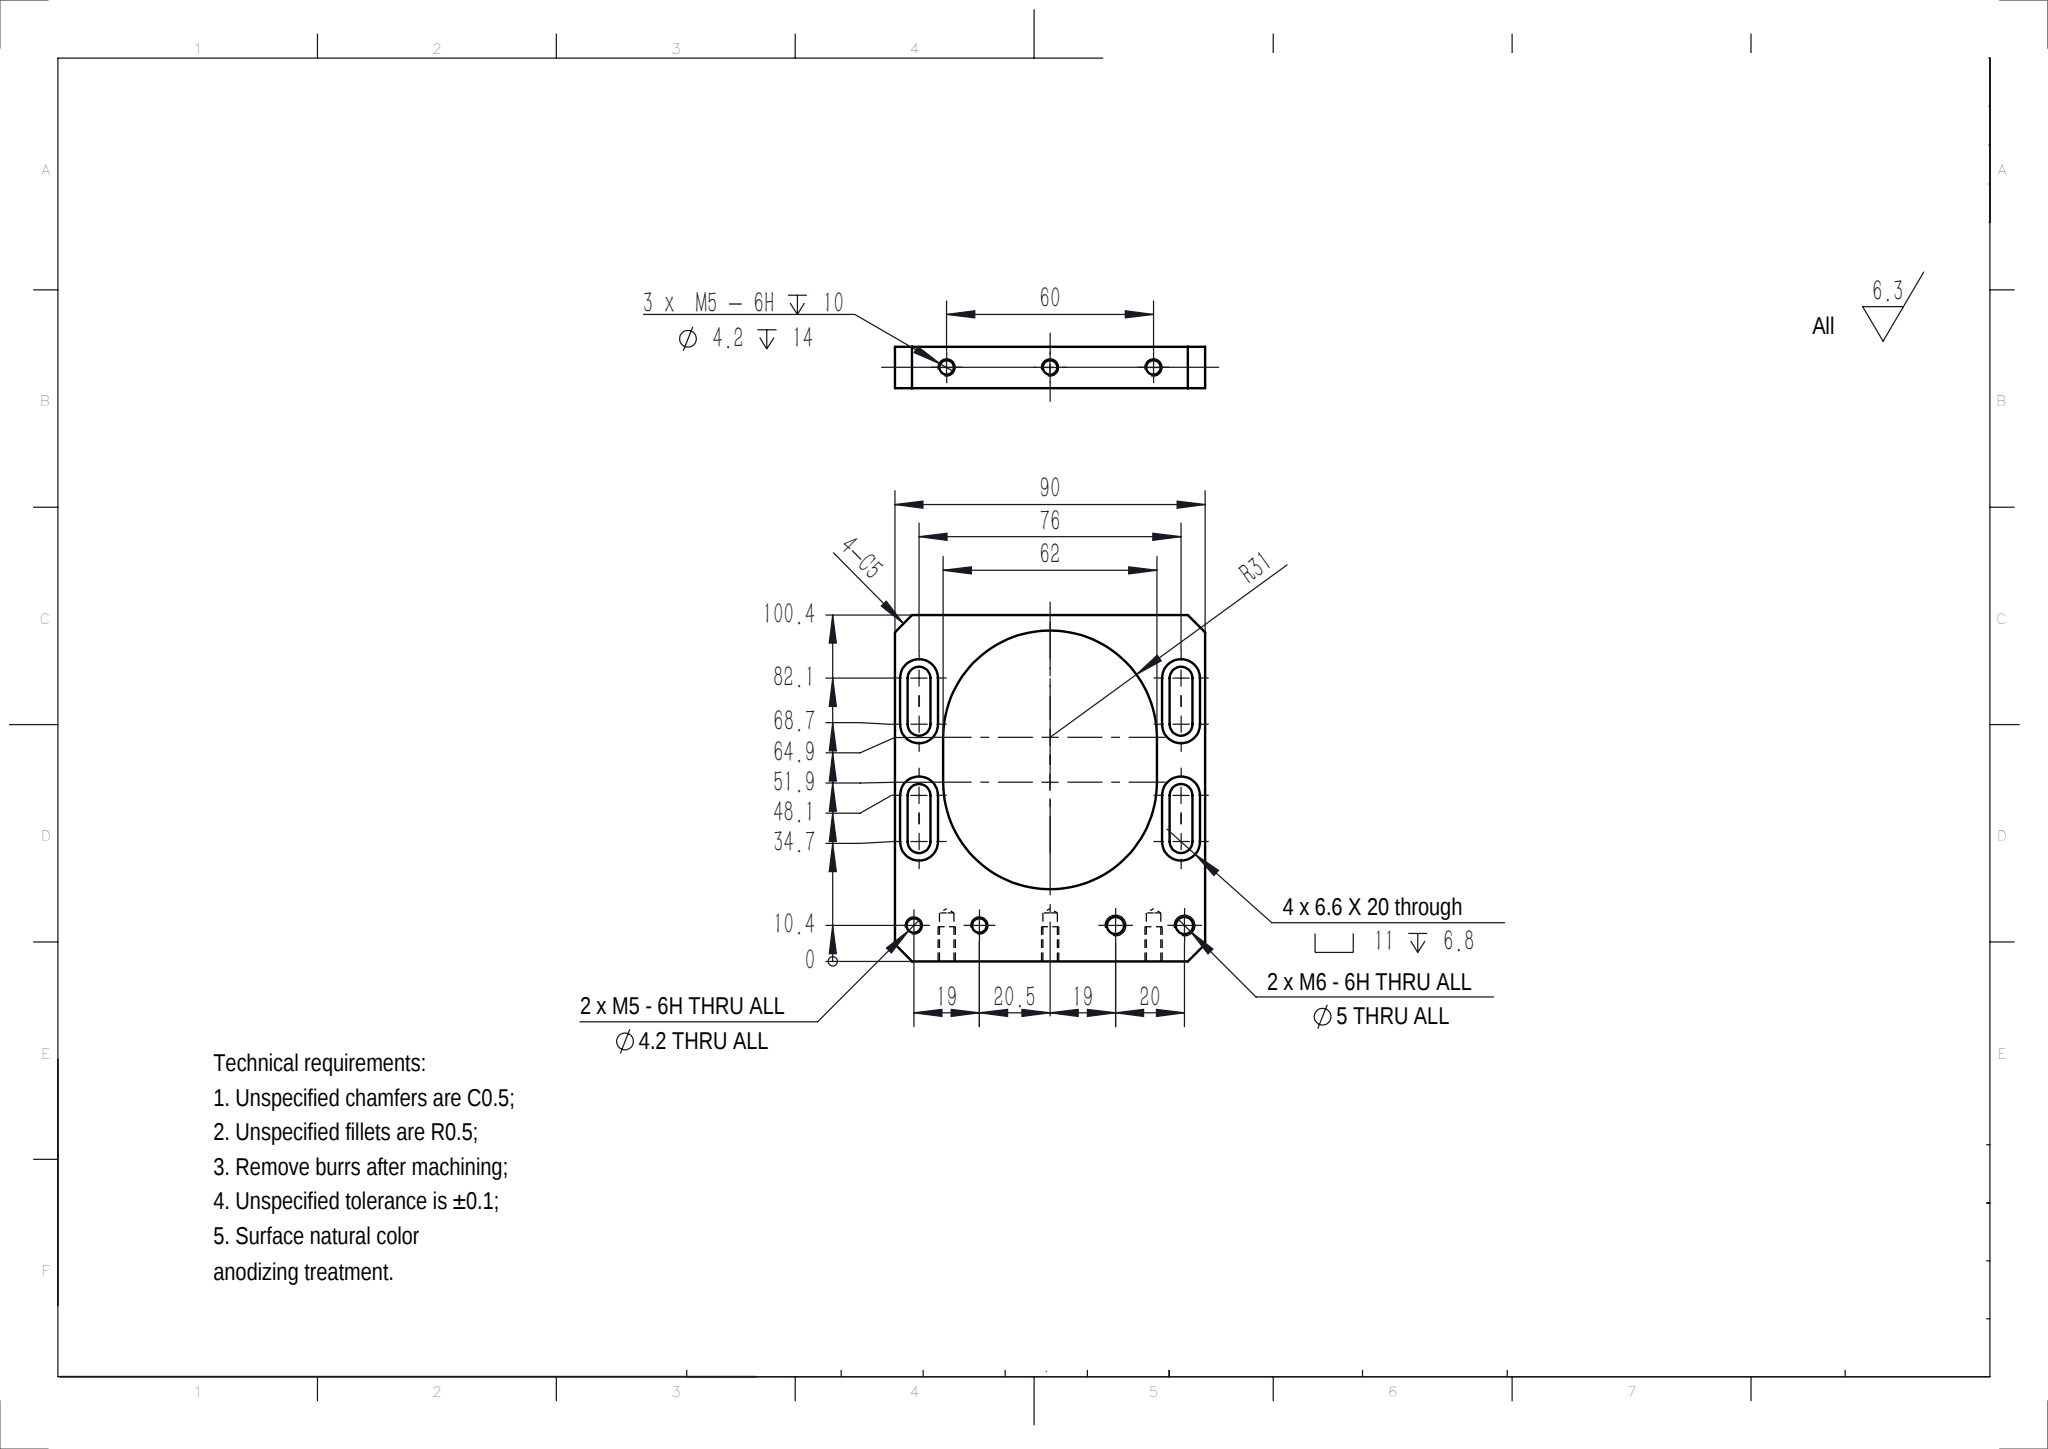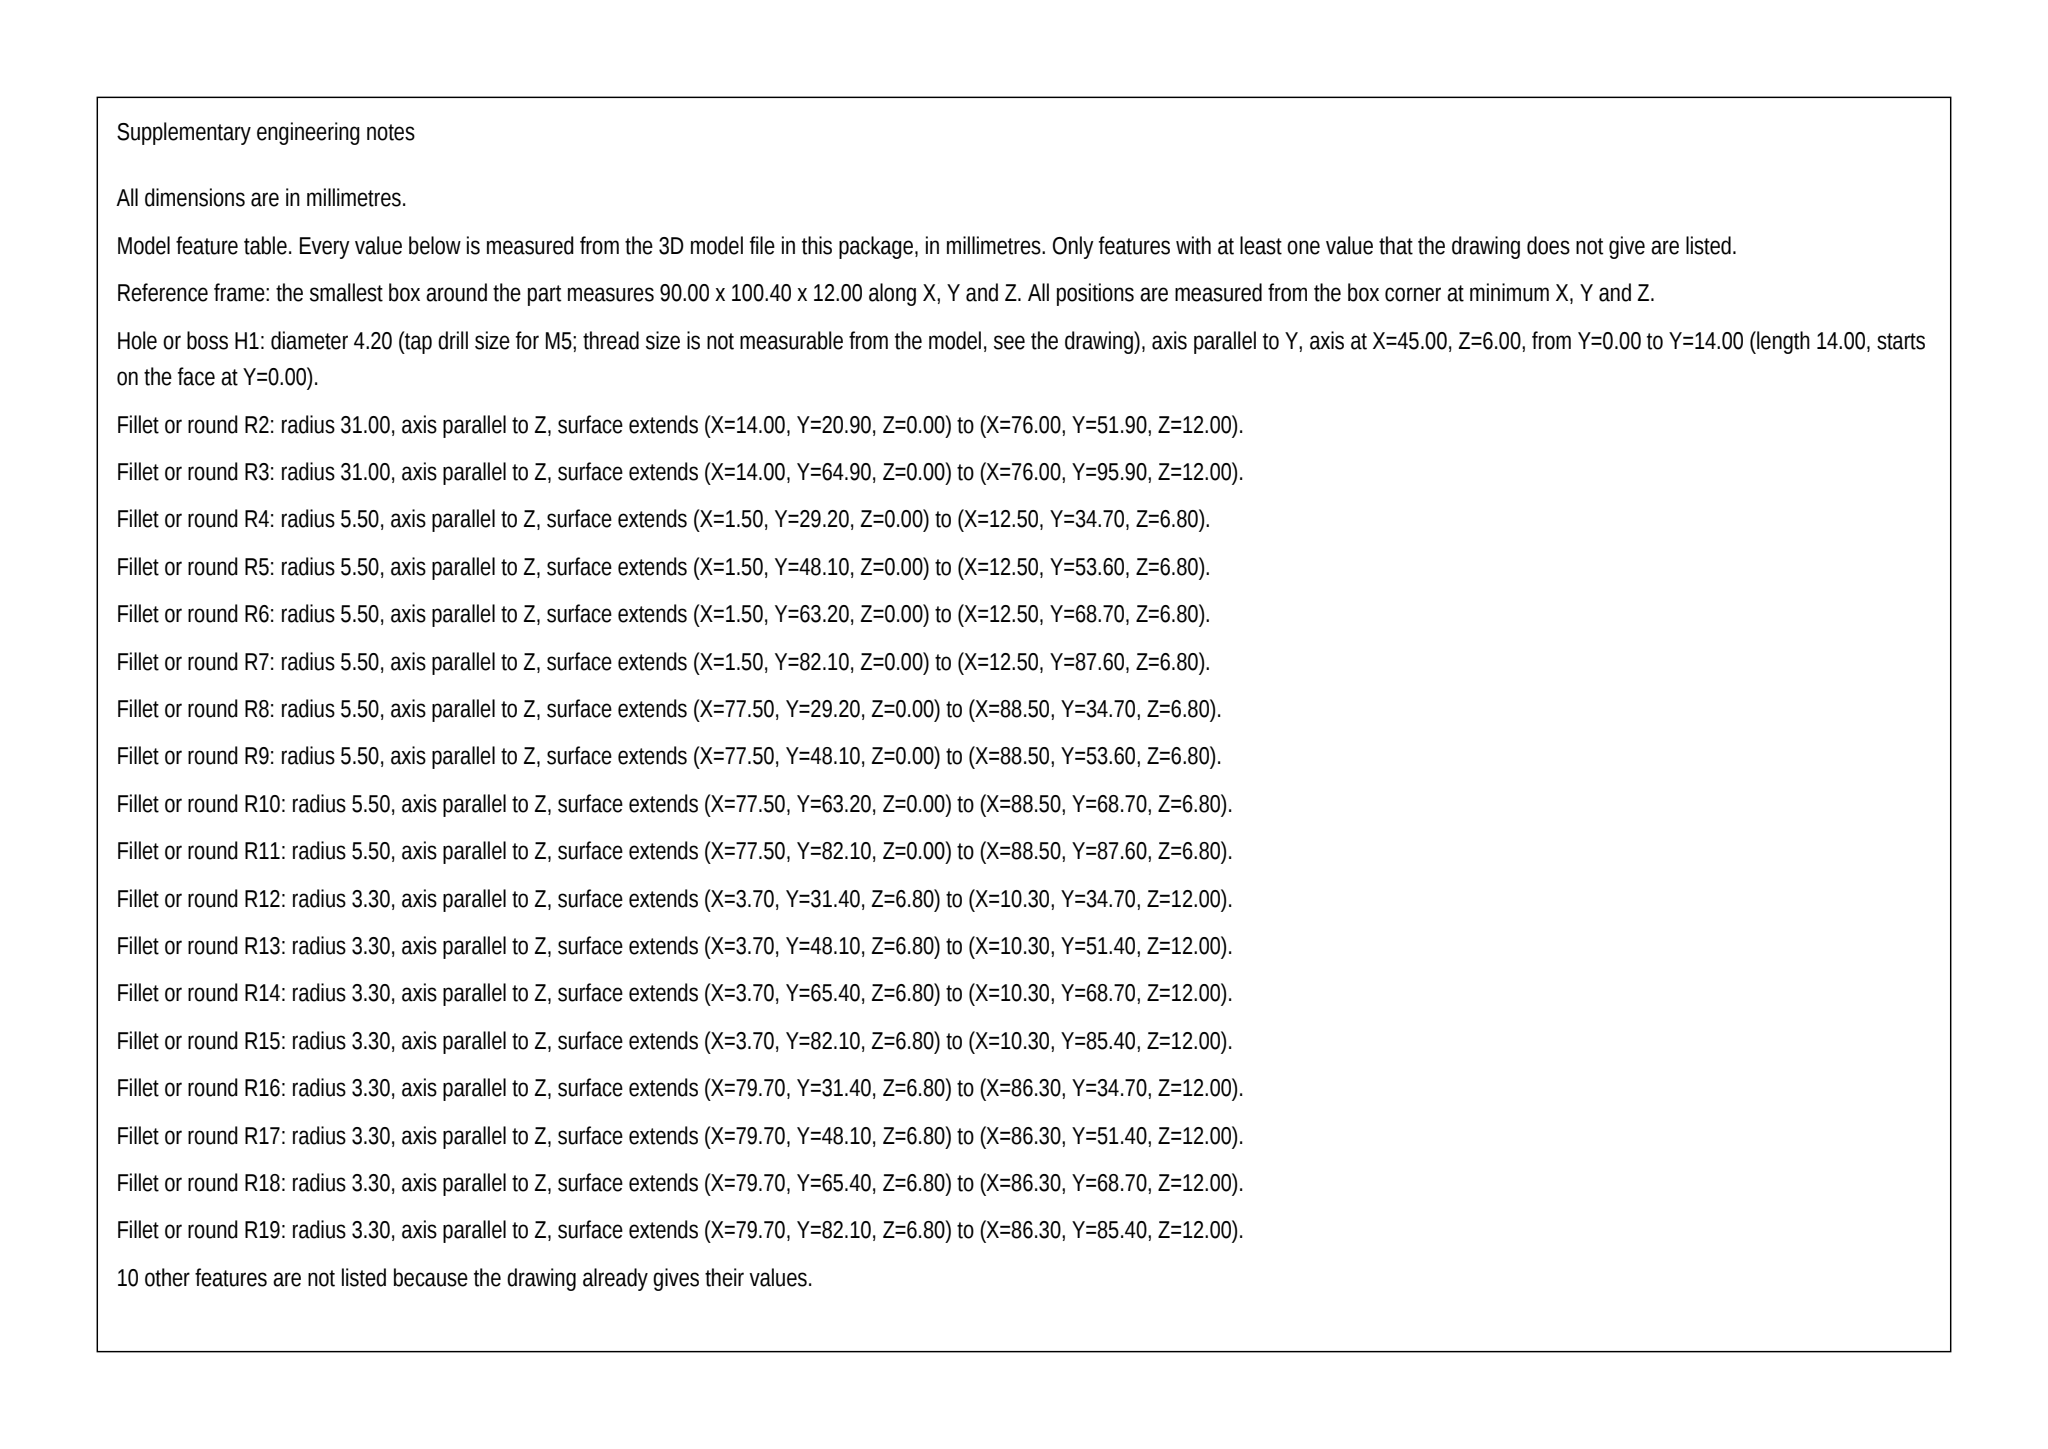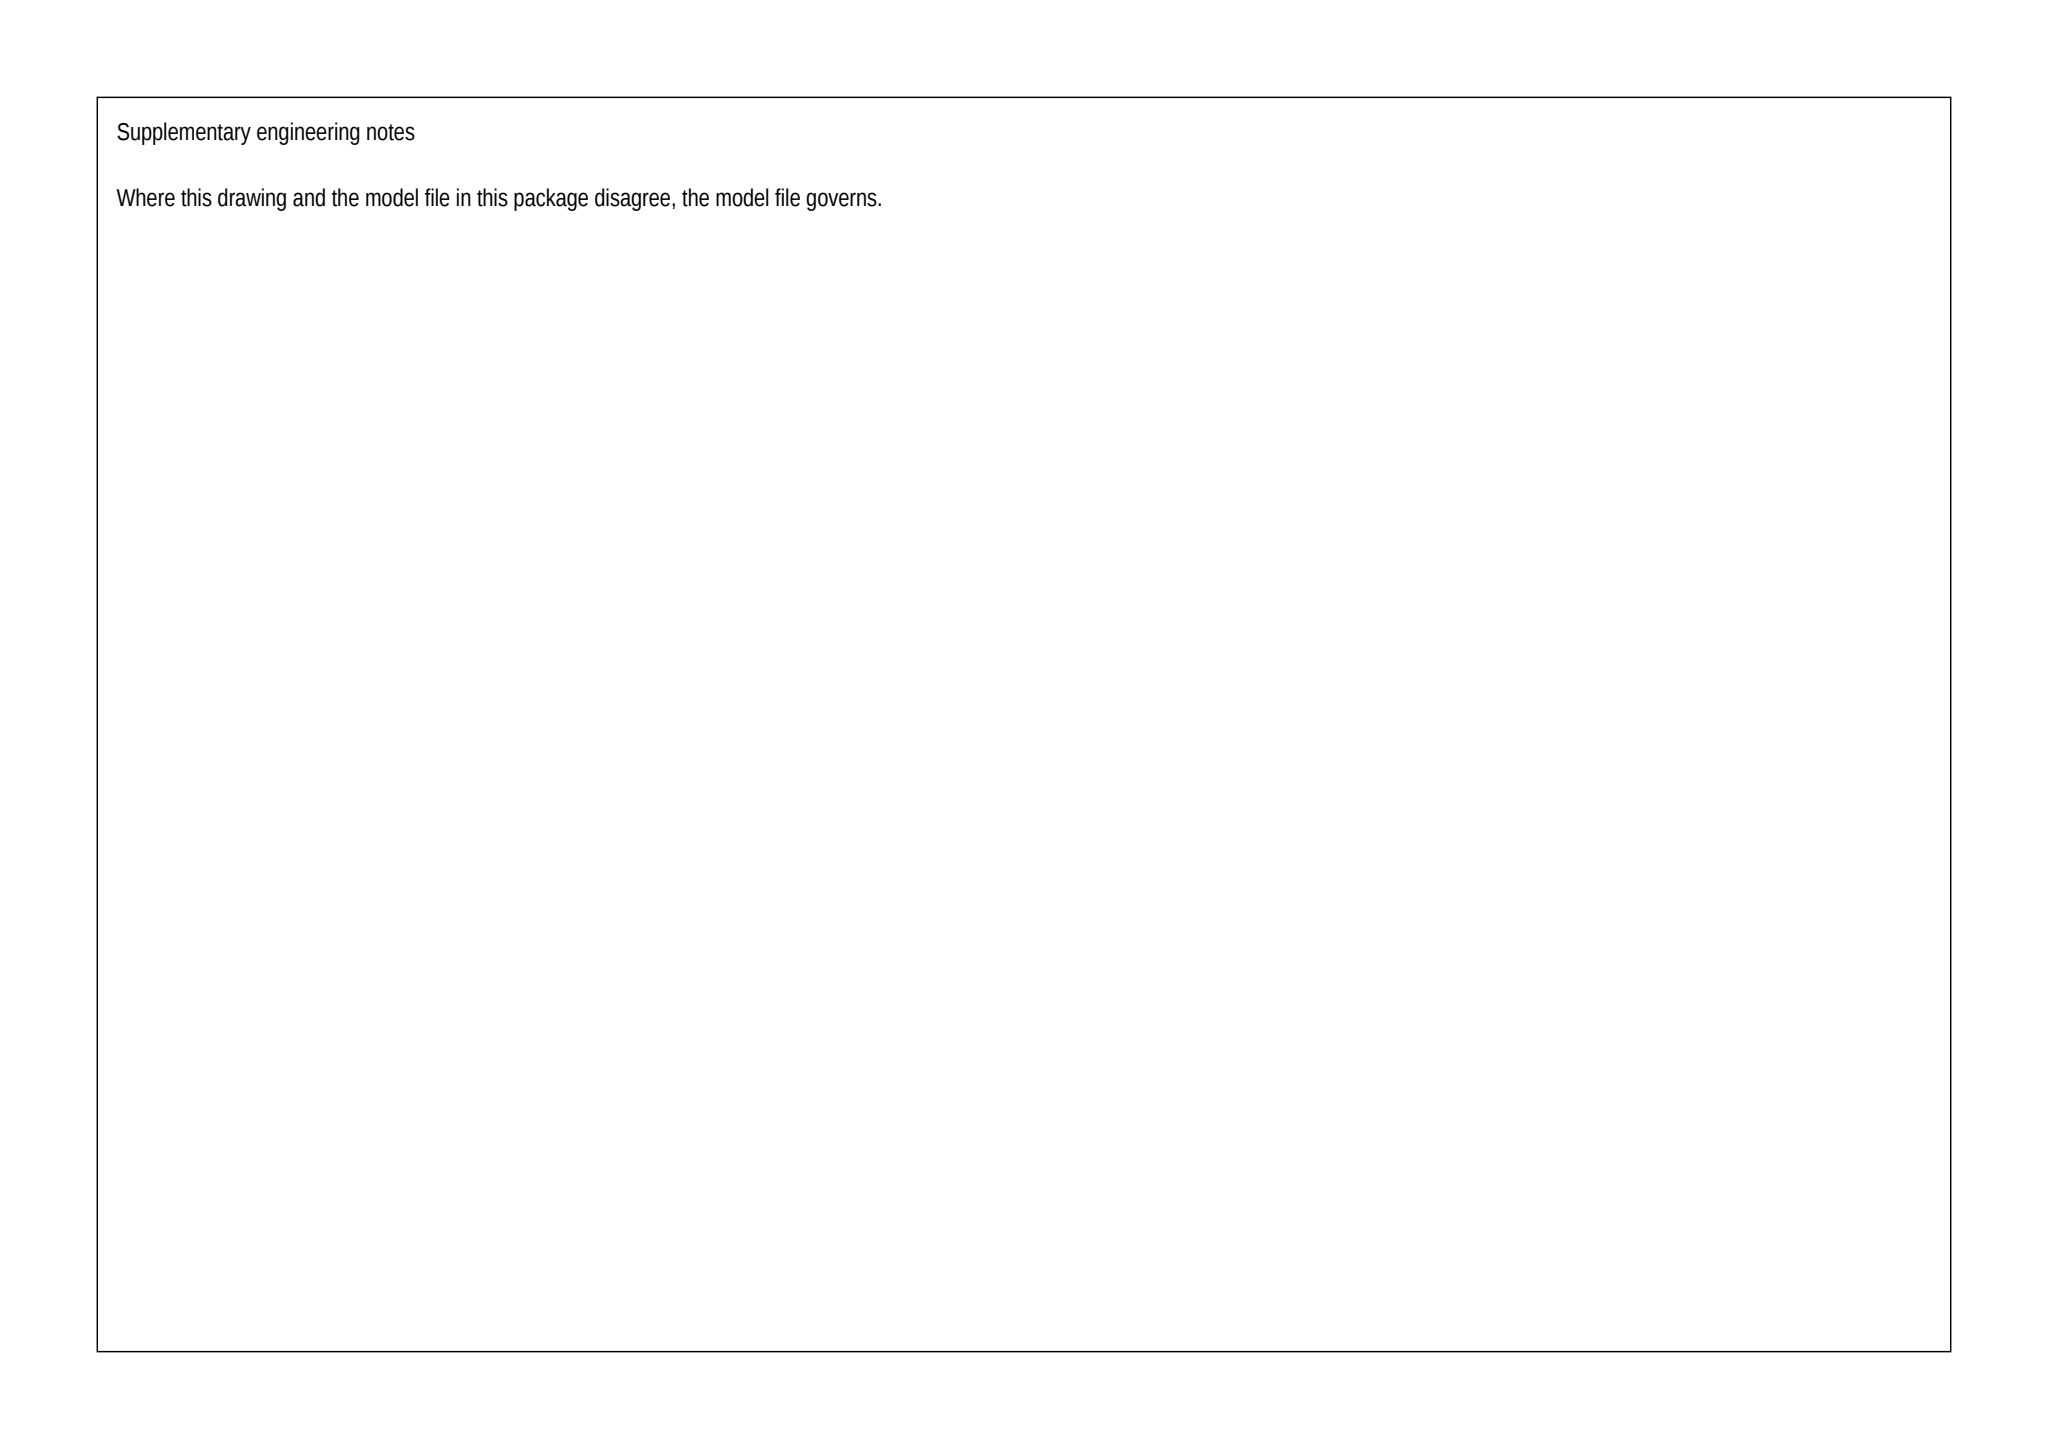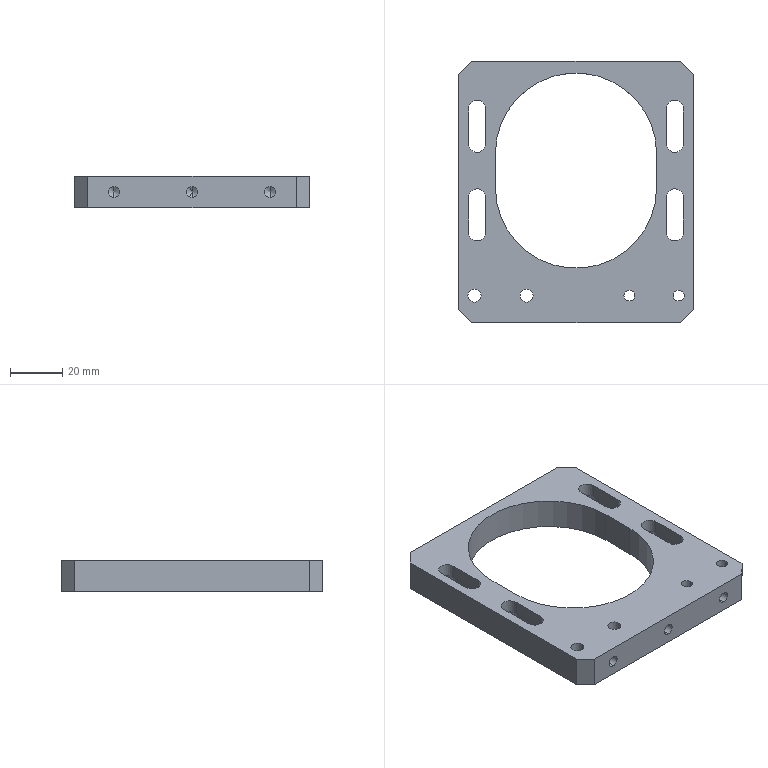Part | SolidWorks | mm | 1 solid | 70 faces | box 90 x 100.4 x 12 mm | volume 51383 mm3 | cylinder 32 | plane 32 | cone 6 | commonest cylinder face diameters 4.2 x10 6.6 x8 11 x8 5 x4 62 x2